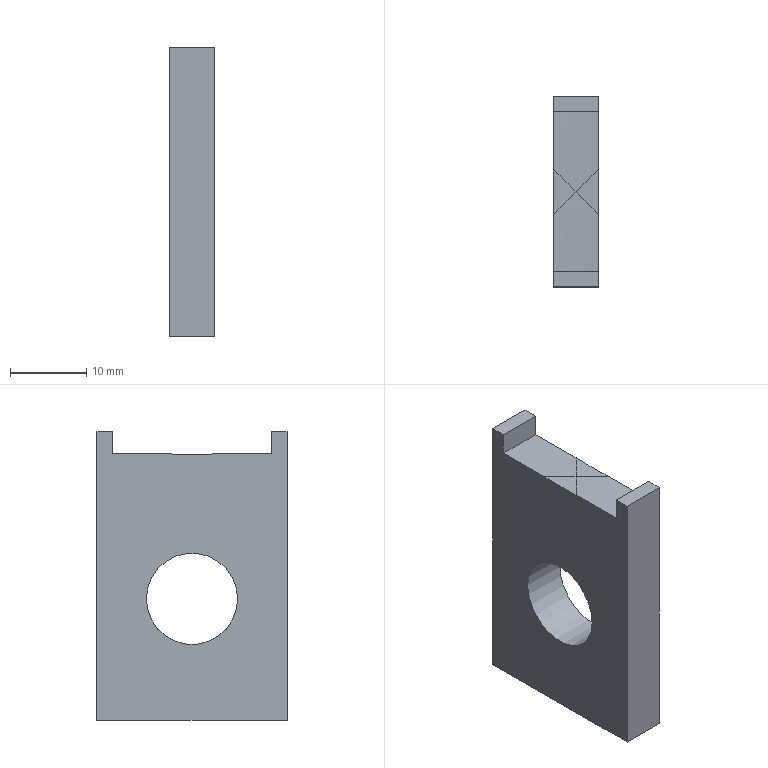Component | NX | PACKING | 1 solid | 14 faces | box 6 x 25 x 38 mm | volume 4646 mm3 | plane 9 | cylinder 5 | commonest cylinder face diameters 152 x4 12 x1
STEP:
#1=CARTESIAN_POINT('',(0.,0.,0.));
#2=DIRECTION('',(0.,0.,1.));
#3=DIRECTION('',(1.,0.,0.));
#4=AXIS2_PLACEMENT_3D('',#1,#2,#3);
#5=CARTESIAN_POINT('',(56.,3.,-75.941));
#6=VERTEX_POINT('',#5);
#7=CARTESIAN_POINT('',(56.,-3.,-75.941));
#8=VERTEX_POINT('',#7);
#9=CARTESIAN_POINT('',(56.,-0.,-0.));
#10=DIRECTION('',(-1.,0.,0.));
#11=DIRECTION('',(0.,-1.,-0.));
#12=AXIS2_PLACEMENT_3D('',#9,#10,#11);
#13=CIRCLE('',#12,76.);
#14=CARTESIAN_POINT('',(62.,-0.,-0.));
#15=DIRECTION('',(-1.,0.,0.));
#16=DIRECTION('',(0.,0.,-1.));
#17=AXIS2_PLACEMENT_3D('',#14,#15,#16);
#18=CYLINDRICAL_SURFACE('',#17,76.);
#19=CARTESIAN_POINT('',(1.571,6.));
#20=DIRECTION('',(1.,0.));
#21=VECTOR('',#20,1.);
#22=LINE('',#19,#21);
#23=(GEOMETRIC_REPRESENTATION_CONTEXT(2)PARAMETRIC_REPRESENTATION_CONTEXT()REPRESENTATION_CONTEXT('',''));
#24=DEFINITIONAL_REPRESENTATION('',(#22),#23);
#25=PCURVE('',#18,#24);
#26=CARTESIAN_POINT('',(56.,-0.,-0.));
#27=DIRECTION('',(-1.,0.,0.));
#28=DIRECTION('',(0.,0.,-1.));
#29=AXIS2_PLACEMENT_3D('',#26,#27,#28);
#30=PLANE('',#29);
#31=CARTESIAN_POINT('',(0.,0.));
#32=DIRECTION('',(0.,1.));
#33=AXIS2_PLACEMENT_2D('',#31,#32);
#34=CIRCLE('',#33,76.);
#35=(GEOMETRIC_REPRESENTATION_CONTEXT(2)PARAMETRIC_REPRESENTATION_CONTEXT()REPRESENTATION_CONTEXT('',''));
#36=DEFINITIONAL_REPRESENTATION('',(#34),#35);
#37=PCURVE('',#30,#36);
#38=SURFACE_CURVE('',#13,(#25,#37),.PCURVE_S1.);
#39=EDGE_CURVE('',#6,#8,#38,.T.);
#40=ORIENTED_EDGE('',*,*,#39,.F.);
#41=CARTESIAN_POINT('',(59.,-0.,-76.));
#42=VERTEX_POINT('',#41);
#43=CARTESIAN_POINT('',(59.,-0.,-0.));
#44=DIRECTION('',(0.7071,0.7071,0.));
#45=DIRECTION('',(-0.7071,0.7071,0.));
#46=AXIS2_PLACEMENT_3D('',#43,#44,#45);
#47=ELLIPSE('',#46,107.48,76.);
#48=CARTESIAN_POINT('',(6.283,3.));
#49=CARTESIAN_POINT('',(6.244,6.));
#50=B_SPLINE_CURVE_WITH_KNOTS('',1,(#48,#49),.UNSPECIFIED.,.F.,.F.,(2,2),(4.712,4.752),.PIECEWISE_BEZIER_KNOTS.);
#51=(GEOMETRIC_REPRESENTATION_CONTEXT(2)PARAMETRIC_REPRESENTATION_CONTEXT()REPRESENTATION_CONTEXT('',''));
#52=DEFINITIONAL_REPRESENTATION('',(#50),#51);
#53=PCURVE('',#18,#52);
#54=CARTESIAN_POINT('',(59.,10.5,-0.));
#55=DIRECTION('',(0.,-1.,0.));
#56=DIRECTION('',(1.,0.,0.));
#57=AXIS2_PLACEMENT_3D('',#54,#55,#56);
#58=CYLINDRICAL_SURFACE('',#57,76.);
#59=CARTESIAN_POINT('',(4.712,10.5));
#60=CARTESIAN_POINT('',(4.673,7.5));
#61=B_SPLINE_CURVE_WITH_KNOTS('',1,(#59,#60),.UNSPECIFIED.,.F.,.F.,(2,2),(4.712,4.752),.PIECEWISE_BEZIER_KNOTS.);
#62=(GEOMETRIC_REPRESENTATION_CONTEXT(2)PARAMETRIC_REPRESENTATION_CONTEXT()REPRESENTATION_CONTEXT('',''));
#63=DEFINITIONAL_REPRESENTATION('',(#61),#62);
#64=PCURVE('',#58,#63);
#65=SURFACE_CURVE('',#47,(#53,#64),.PCURVE_S1.);
#66=EDGE_CURVE('',#42,#6,#65,.T.);
#67=ORIENTED_EDGE('',*,*,#66,.F.);
#68=CARTESIAN_POINT('',(59.,-0.,-0.));
#69=DIRECTION('',(0.7071,-0.7071,0.));
#70=DIRECTION('',(-0.7071,-0.7071,0.));
#71=AXIS2_PLACEMENT_3D('',#68,#69,#70);
#72=ELLIPSE('',#71,107.48,76.);
#73=CARTESIAN_POINT('',(6.323,6.));
#74=CARTESIAN_POINT('',(6.283,3.));
#75=B_SPLINE_CURVE_WITH_KNOTS('',1,(#73,#74),.UNSPECIFIED.,.F.,.F.,(2,2),(1.531,1.571),.PIECEWISE_BEZIER_KNOTS.);
#76=(GEOMETRIC_REPRESENTATION_CONTEXT(2)PARAMETRIC_REPRESENTATION_CONTEXT()REPRESENTATION_CONTEXT('',''));
#77=DEFINITIONAL_REPRESENTATION('',(#75),#76);
#78=PCURVE('',#18,#77);
#79=CARTESIAN_POINT('',(59.,10.5,-0.));
#80=DIRECTION('',(0.,-1.,0.));
#81=DIRECTION('',(1.,0.,0.));
#82=AXIS2_PLACEMENT_3D('',#79,#80,#81);
#83=CYLINDRICAL_SURFACE('',#82,76.);
#84=CARTESIAN_POINT('',(4.673,13.5));
#85=CARTESIAN_POINT('',(4.712,10.5));
#86=B_SPLINE_CURVE_WITH_KNOTS('',1,(#84,#85),.UNSPECIFIED.,.F.,.F.,(2,2),(1.531,1.571),.PIECEWISE_BEZIER_KNOTS.);
#87=(GEOMETRIC_REPRESENTATION_CONTEXT(2)PARAMETRIC_REPRESENTATION_CONTEXT()REPRESENTATION_CONTEXT('',''));
#88=DEFINITIONAL_REPRESENTATION('',(#86),#87);
#89=PCURVE('',#83,#88);
#90=SURFACE_CURVE('',#72,(#78,#89),.PCURVE_S1.);
#91=EDGE_CURVE('',#8,#42,#90,.T.);
#92=ORIENTED_EDGE('',*,*,#91,.F.);
#93=EDGE_LOOP('',(#40,#67,#92));
#94=FACE_BOUND('',#93,.F.);
#95=ADVANCED_FACE('',(#94),#18,.F.);
#96=CARTESIAN_POINT('',(56.,12.5,-111.));
#97=VERTEX_POINT('',#96);
#98=CARTESIAN_POINT('',(56.,12.5,-73.));
#99=VERTEX_POINT('',#98);
#100=CARTESIAN_POINT('',(56.,12.5,-111.));
#101=DIRECTION('',(0.,0.,1.));
#102=VECTOR('',#101,1.);
#103=LINE('',#100,#102);
#104=CARTESIAN_POINT('',(62.,12.5,-111.));
#105=DIRECTION('',(0.,-1.,0.));
#106=DIRECTION('',(0.,-0.,-1.));
#107=AXIS2_PLACEMENT_3D('',#104,#105,#106);
#108=PLANE('',#107);
#109=CARTESIAN_POINT('',(0.,-6.));
#110=DIRECTION('',(-1.,0.));
#111=VECTOR('',#110,1.);
#112=LINE('',#109,#111);
#113=(GEOMETRIC_REPRESENTATION_CONTEXT(2)PARAMETRIC_REPRESENTATION_CONTEXT()REPRESENTATION_CONTEXT('',''));
#114=DEFINITIONAL_REPRESENTATION('',(#112),#113);
#115=PCURVE('',#108,#114);
#116=CARTESIAN_POINT('',(111.,-12.5));
#117=DIRECTION('',(-1.,-0.));
#118=VECTOR('',#117,1.);
#119=LINE('',#116,#118);
#120=(GEOMETRIC_REPRESENTATION_CONTEXT(2)PARAMETRIC_REPRESENTATION_CONTEXT()REPRESENTATION_CONTEXT('',''));
#121=DEFINITIONAL_REPRESENTATION('',(#119),#120);
#122=PCURVE('',#30,#121);
#123=SURFACE_CURVE('',#103,(#115,#122),.PCURVE_S1.);
#124=EDGE_CURVE('',#97,#99,#123,.T.);
#125=ORIENTED_EDGE('',*,*,#124,.T.);
#126=CARTESIAN_POINT('',(62.,12.5,-73.));
#127=VERTEX_POINT('',#126);
#128=CARTESIAN_POINT('',(62.,12.5,-73.));
#129=DIRECTION('',(-1.,0.,0.));
#130=VECTOR('',#129,1.);
#131=LINE('',#128,#130);
#132=CARTESIAN_POINT('',(-38.,0.));
#133=DIRECTION('',(0.,-1.));
#134=VECTOR('',#133,1.);
#135=LINE('',#132,#134);
#136=(GEOMETRIC_REPRESENTATION_CONTEXT(2)PARAMETRIC_REPRESENTATION_CONTEXT()REPRESENTATION_CONTEXT('',''));
#137=DEFINITIONAL_REPRESENTATION('',(#135),#136);
#138=PCURVE('',#108,#137);
#139=CARTESIAN_POINT('',(62.,12.5,-73.));
#140=DIRECTION('',(0.,-0.,-1.));
#141=DIRECTION('',(0.,1.,-0.));
#142=AXIS2_PLACEMENT_3D('',#139,#140,#141);
#143=PLANE('',#142);
#144=CARTESIAN_POINT('',(0.,0.));
#145=DIRECTION('',(0.,-1.));
#146=VECTOR('',#145,1.);
#147=LINE('',#144,#146);
#148=(GEOMETRIC_REPRESENTATION_CONTEXT(2)PARAMETRIC_REPRESENTATION_CONTEXT()REPRESENTATION_CONTEXT('',''));
#149=DEFINITIONAL_REPRESENTATION('',(#147),#148);
#150=PCURVE('',#143,#149);
#151=SURFACE_CURVE('',#131,(#138,#150),.PCURVE_S1.);
#152=EDGE_CURVE('',#127,#99,#151,.T.);
#153=ORIENTED_EDGE('',*,*,#152,.F.);
#154=CARTESIAN_POINT('',(62.,12.5,-111.));
#155=VERTEX_POINT('',#154);
#156=CARTESIAN_POINT('',(62.,12.5,-111.));
#157=DIRECTION('',(0.,0.,1.));
#158=VECTOR('',#157,1.);
#159=LINE('',#156,#158);
#160=CARTESIAN_POINT('',(0.,0.));
#161=DIRECTION('',(-1.,0.));
#162=VECTOR('',#161,1.);
#163=LINE('',#160,#162);
#164=(GEOMETRIC_REPRESENTATION_CONTEXT(2)PARAMETRIC_REPRESENTATION_CONTEXT()REPRESENTATION_CONTEXT('',''));
#165=DEFINITIONAL_REPRESENTATION('',(#163),#164);
#166=PCURVE('',#108,#165);
#167=CARTESIAN_POINT('',(62.,-0.,-0.));
#168=DIRECTION('',(-1.,0.,0.));
#169=DIRECTION('',(0.,0.,-1.));
#170=AXIS2_PLACEMENT_3D('',#167,#168,#169);
#171=PLANE('',#170);
#172=CARTESIAN_POINT('',(111.,-12.5));
#173=DIRECTION('',(-1.,-0.));
#174=VECTOR('',#173,1.);
#175=LINE('',#172,#174);
#176=(GEOMETRIC_REPRESENTATION_CONTEXT(2)PARAMETRIC_REPRESENTATION_CONTEXT()REPRESENTATION_CONTEXT('',''));
#177=DEFINITIONAL_REPRESENTATION('',(#175),#176);
#178=PCURVE('',#171,#177);
#179=SURFACE_CURVE('',#159,(#166,#178),.PCURVE_S1.);
#180=EDGE_CURVE('',#155,#127,#179,.T.);
#181=ORIENTED_EDGE('',*,*,#180,.F.);
#182=CARTESIAN_POINT('',(62.,12.5,-111.));
#183=DIRECTION('',(-1.,0.,0.));
#184=VECTOR('',#183,1.);
#185=LINE('',#182,#184);
#186=CARTESIAN_POINT('',(0.,0.));
#187=DIRECTION('',(0.,-1.));
#188=VECTOR('',#187,1.);
#189=LINE('',#186,#188);
#190=(GEOMETRIC_REPRESENTATION_CONTEXT(2)PARAMETRIC_REPRESENTATION_CONTEXT()REPRESENTATION_CONTEXT('',''));
#191=DEFINITIONAL_REPRESENTATION('',(#189),#190);
#192=PCURVE('',#108,#191);
#193=CARTESIAN_POINT('',(62.,-0.,-111.));
#194=DIRECTION('',(0.,0.,1.));
#195=DIRECTION('',(-1.,0.,0.));
#196=AXIS2_PLACEMENT_3D('',#193,#194,#195);
#197=PLANE('',#196);
#198=CARTESIAN_POINT('',(0.,-12.5));
#199=DIRECTION('',(1.,0.));
#200=VECTOR('',#199,1.);
#201=LINE('',#198,#200);
#202=(GEOMETRIC_REPRESENTATION_CONTEXT(2)PARAMETRIC_REPRESENTATION_CONTEXT()REPRESENTATION_CONTEXT('',''));
#203=DEFINITIONAL_REPRESENTATION('',(#201),#202);
#204=PCURVE('',#197,#203);
#205=SURFACE_CURVE('',#185,(#192,#204),.PCURVE_S1.);
#206=EDGE_CURVE('',#155,#97,#205,.T.);
#207=ORIENTED_EDGE('',*,*,#206,.T.);
#208=EDGE_LOOP('',(#125,#153,#181,#207));
#209=FACE_BOUND('',#208,.T.);
#210=ADVANCED_FACE('',(#209),#108,.F.);
#211=CARTESIAN_POINT('',(56.,10.5,-73.));
#212=VERTEX_POINT('',#211);
#213=CARTESIAN_POINT('',(56.,12.5,-73.));
#214=DIRECTION('',(0.,-1.,0.));
#215=VECTOR('',#214,1.);
#216=LINE('',#213,#215);
#217=CARTESIAN_POINT('',(0.,-6.));
#218=DIRECTION('',(-1.,0.));
#219=VECTOR('',#218,1.);
#220=LINE('',#217,#219);
#221=(GEOMETRIC_REPRESENTATION_CONTEXT(2)PARAMETRIC_REPRESENTATION_CONTEXT()REPRESENTATION_CONTEXT('',''));
#222=DEFINITIONAL_REPRESENTATION('',(#220),#221);
#223=PCURVE('',#143,#222);
#224=CARTESIAN_POINT('',(73.,-12.5));
#225=DIRECTION('',(-0.,1.));
#226=VECTOR('',#225,1.);
#227=LINE('',#224,#226);
#228=(GEOMETRIC_REPRESENTATION_CONTEXT(2)PARAMETRIC_REPRESENTATION_CONTEXT()REPRESENTATION_CONTEXT('',''));
#229=DEFINITIONAL_REPRESENTATION('',(#227),#228);
#230=PCURVE('',#30,#229);
#231=SURFACE_CURVE('',#216,(#223,#230),.PCURVE_S1.);
#232=EDGE_CURVE('',#99,#212,#231,.T.);
#233=ORIENTED_EDGE('',*,*,#232,.T.);
#234=CARTESIAN_POINT('',(62.,10.5,-73.));
#235=VERTEX_POINT('',#234);
#236=CARTESIAN_POINT('',(62.,10.5,-73.));
#237=DIRECTION('',(-1.,0.,0.));
#238=VECTOR('',#237,1.);
#239=LINE('',#236,#238);
#240=CARTESIAN_POINT('',(-2.,0.));
#241=DIRECTION('',(0.,-1.));
#242=VECTOR('',#241,1.);
#243=LINE('',#240,#242);
#244=(GEOMETRIC_REPRESENTATION_CONTEXT(2)PARAMETRIC_REPRESENTATION_CONTEXT()REPRESENTATION_CONTEXT('',''));
#245=DEFINITIONAL_REPRESENTATION('',(#243),#244);
#246=PCURVE('',#143,#245);
#247=CARTESIAN_POINT('',(62.,10.5,-73.));
#248=DIRECTION('',(0.,1.,0.));
#249=DIRECTION('',(0.,0.,1.));
#250=AXIS2_PLACEMENT_3D('',#247,#248,#249);
#251=PLANE('',#250);
#252=CARTESIAN_POINT('',(0.,0.));
#253=DIRECTION('',(0.,-1.));
#254=VECTOR('',#253,1.);
#255=LINE('',#252,#254);
#256=(GEOMETRIC_REPRESENTATION_CONTEXT(2)PARAMETRIC_REPRESENTATION_CONTEXT()REPRESENTATION_CONTEXT('',''));
#257=DEFINITIONAL_REPRESENTATION('',(#255),#256);
#258=PCURVE('',#251,#257);
#259=SURFACE_CURVE('',#239,(#246,#258),.PCURVE_S1.);
#260=EDGE_CURVE('',#235,#212,#259,.T.);
#261=ORIENTED_EDGE('',*,*,#260,.F.);
#262=CARTESIAN_POINT('',(62.,12.5,-73.));
#263=DIRECTION('',(0.,-1.,0.));
#264=VECTOR('',#263,1.);
#265=LINE('',#262,#264);
#266=CARTESIAN_POINT('',(0.,0.));
#267=DIRECTION('',(-1.,0.));
#268=VECTOR('',#267,1.);
#269=LINE('',#266,#268);
#270=(GEOMETRIC_REPRESENTATION_CONTEXT(2)PARAMETRIC_REPRESENTATION_CONTEXT()REPRESENTATION_CONTEXT('',''));
#271=DEFINITIONAL_REPRESENTATION('',(#269),#270);
#272=PCURVE('',#143,#271);
#273=CARTESIAN_POINT('',(73.,-12.5));
#274=DIRECTION('',(-0.,1.));
#275=VECTOR('',#274,1.);
#276=LINE('',#273,#275);
#277=(GEOMETRIC_REPRESENTATION_CONTEXT(2)PARAMETRIC_REPRESENTATION_CONTEXT()REPRESENTATION_CONTEXT('',''));
#278=DEFINITIONAL_REPRESENTATION('',(#276),#277);
#279=PCURVE('',#171,#278);
#280=SURFACE_CURVE('',#265,(#272,#279),.PCURVE_S1.);
#281=EDGE_CURVE('',#127,#235,#280,.T.);
#282=ORIENTED_EDGE('',*,*,#281,.F.);
#283=ORIENTED_EDGE('',*,*,#152,.T.);
#284=EDGE_LOOP('',(#233,#261,#282,#283));
#285=FACE_BOUND('',#284,.T.);
#286=ADVANCED_FACE('',(#285),#143,.F.);
#287=CARTESIAN_POINT('',(56.,10.5,-75.941));
#288=VERTEX_POINT('',#287);
#289=CARTESIAN_POINT('',(56.,10.5,-73.));
#290=DIRECTION('',(0.,0.,-1.));
#291=VECTOR('',#290,1.);
#292=LINE('',#289,#291);
#293=CARTESIAN_POINT('',(0.,-6.));
#294=DIRECTION('',(-1.,0.));
#295=VECTOR('',#294,1.);
#296=LINE('',#293,#295);
#297=(GEOMETRIC_REPRESENTATION_CONTEXT(2)PARAMETRIC_REPRESENTATION_CONTEXT()REPRESENTATION_CONTEXT('',''));
#298=DEFINITIONAL_REPRESENTATION('',(#296),#297);
#299=PCURVE('',#251,#298);
#300=CARTESIAN_POINT('',(73.,-10.5));
#301=DIRECTION('',(1.,0.));
#302=VECTOR('',#301,1.);
#303=LINE('',#300,#302);
#304=(GEOMETRIC_REPRESENTATION_CONTEXT(2)PARAMETRIC_REPRESENTATION_CONTEXT()REPRESENTATION_CONTEXT('',''));
#305=DEFINITIONAL_REPRESENTATION('',(#303),#304);
#306=PCURVE('',#30,#305);
#307=SURFACE_CURVE('',#292,(#299,#306),.PCURVE_S1.);
#308=EDGE_CURVE('',#212,#288,#307,.T.);
#309=ORIENTED_EDGE('',*,*,#308,.T.);
#310=CARTESIAN_POINT('',(62.,10.5,-75.941));
#311=VERTEX_POINT('',#310);
#312=CARTESIAN_POINT('',(59.,10.5,-0.));
#313=DIRECTION('',(0.,-1.,0.));
#314=DIRECTION('',(1.,0.,0.));
#315=AXIS2_PLACEMENT_3D('',#312,#313,#314);
#316=CIRCLE('',#315,76.);
#317=CARTESIAN_POINT('',(73.,73.));
#318=CARTESIAN_POINT('',(204.636,73.));
#319=CARTESIAN_POINT('',(138.818,-41.));
#320=CARTESIAN_POINT('',(73.,-155.));
#321=CARTESIAN_POINT('',(7.182,-41.));
#322=CARTESIAN_POINT('',(-58.636,73.));
#323=CARTESIAN_POINT('',(73.,73.));
#324=(BOUNDED_CURVE()B_SPLINE_CURVE(2,(#317,#318,#319,#320,#321,#322,#323),.UNSPECIFIED.,.T.,.F.)B_SPLINE_CURVE_WITH_KNOTS((1,2,2,2,2,1),(-2.094,0.,2.094,4.189,6.283,8.378),.UNSPECIFIED.)CURVE()GEOMETRIC_REPRESENTATION_ITEM()RATIONAL_B_SPLINE_CURVE((1.,0.5,1.,0.5,1.,0.5,1.))REPRESENTATION_ITEM(''));
#325=(GEOMETRIC_REPRESENTATION_CONTEXT(2)PARAMETRIC_REPRESENTATION_CONTEXT()REPRESENTATION_CONTEXT('',''));
#326=DEFINITIONAL_REPRESENTATION('',(#324),#325);
#327=PCURVE('',#251,#326);
#328=CARTESIAN_POINT('',(0.,0.));
#329=DIRECTION('',(1.,0.));
#330=VECTOR('',#329,1.);
#331=LINE('',#328,#330);
#332=(GEOMETRIC_REPRESENTATION_CONTEXT(2)PARAMETRIC_REPRESENTATION_CONTEXT()REPRESENTATION_CONTEXT('',''));
#333=DEFINITIONAL_REPRESENTATION('',(#331),#332);
#334=PCURVE('',#58,#333);
#335=SURFACE_CURVE('',#316,(#327,#334),.PCURVE_S1.);
#336=EDGE_CURVE('',#288,#311,#335,.T.);
#337=ORIENTED_EDGE('',*,*,#336,.T.);
#338=CARTESIAN_POINT('',(62.,10.5,-73.));
#339=DIRECTION('',(0.,0.,-1.));
#340=VECTOR('',#339,1.);
#341=LINE('',#338,#340);
#342=CARTESIAN_POINT('',(0.,0.));
#343=DIRECTION('',(-1.,0.));
#344=VECTOR('',#343,1.);
#345=LINE('',#342,#344);
#346=(GEOMETRIC_REPRESENTATION_CONTEXT(2)PARAMETRIC_REPRESENTATION_CONTEXT()REPRESENTATION_CONTEXT('',''));
#347=DEFINITIONAL_REPRESENTATION('',(#345),#346);
#348=PCURVE('',#251,#347);
#349=CARTESIAN_POINT('',(73.,-10.5));
#350=DIRECTION('',(1.,0.));
#351=VECTOR('',#350,1.);
#352=LINE('',#349,#351);
#353=(GEOMETRIC_REPRESENTATION_CONTEXT(2)PARAMETRIC_REPRESENTATION_CONTEXT()REPRESENTATION_CONTEXT('',''));
#354=DEFINITIONAL_REPRESENTATION('',(#352),#353);
#355=PCURVE('',#171,#354);
#356=SURFACE_CURVE('',#341,(#348,#355),.PCURVE_S1.);
#357=EDGE_CURVE('',#235,#311,#356,.T.);
#358=ORIENTED_EDGE('',*,*,#357,.F.);
#359=ORIENTED_EDGE('',*,*,#260,.T.);
#360=EDGE_LOOP('',(#309,#337,#358,#359));
#361=FACE_BOUND('',#360,.T.);
#362=ADVANCED_FACE('',(#361),#251,.F.);
#363=CARTESIAN_POINT('',(62.,3.,-75.941));
#364=VERTEX_POINT('',#363);
#365=CARTESIAN_POINT('',(62.,-3.,-75.941));
#366=VERTEX_POINT('',#365);
#367=CARTESIAN_POINT('',(62.,-0.,-0.));
#368=DIRECTION('',(-1.,0.,0.));
#369=DIRECTION('',(0.,-1.,-0.));
#370=AXIS2_PLACEMENT_3D('',#367,#368,#369);
#371=CIRCLE('',#370,76.);
#372=CARTESIAN_POINT('',(62.,-0.,-0.));
#373=DIRECTION('',(-1.,0.,0.));
#374=DIRECTION('',(0.,0.,-1.));
#375=AXIS2_PLACEMENT_3D('',#372,#373,#374);
#376=CYLINDRICAL_SURFACE('',#375,76.);
#377=CARTESIAN_POINT('',(1.571,0.));
#378=DIRECTION('',(1.,0.));
#379=VECTOR('',#378,1.);
#380=LINE('',#377,#379);
#381=(GEOMETRIC_REPRESENTATION_CONTEXT(2)PARAMETRIC_REPRESENTATION_CONTEXT()REPRESENTATION_CONTEXT('',''));
#382=DEFINITIONAL_REPRESENTATION('',(#380),#381);
#383=PCURVE('',#376,#382);
#384=CARTESIAN_POINT('',(0.,0.));
#385=DIRECTION('',(0.,1.));
#386=AXIS2_PLACEMENT_2D('',#384,#385);
#387=CIRCLE('',#386,76.);
#388=(GEOMETRIC_REPRESENTATION_CONTEXT(2)PARAMETRIC_REPRESENTATION_CONTEXT()REPRESENTATION_CONTEXT('',''));
#389=DEFINITIONAL_REPRESENTATION('',(#387),#388);
#390=PCURVE('',#171,#389);
#391=SURFACE_CURVE('',#371,(#383,#390),.PCURVE_S1.);
#392=EDGE_CURVE('',#364,#366,#391,.T.);
#393=ORIENTED_EDGE('',*,*,#392,.T.);
#394=CARTESIAN_POINT('',(59.,-0.,-0.));
#395=DIRECTION('',(-0.7071,-0.7071,0.));
#396=DIRECTION('',(-0.7071,0.7071,0.));
#397=AXIS2_PLACEMENT_3D('',#394,#395,#396);
#398=ELLIPSE('',#397,107.48,76.);
#399=CARTESIAN_POINT('',(6.283,3.));
#400=CARTESIAN_POINT('',(6.323,-0.));
#401=B_SPLINE_CURVE_WITH_KNOTS('',1,(#399,#400),.UNSPECIFIED.,.F.,.F.,(2,2),(1.571,1.61),.PIECEWISE_BEZIER_KNOTS.);
#402=(GEOMETRIC_REPRESENTATION_CONTEXT(2)PARAMETRIC_REPRESENTATION_CONTEXT()REPRESENTATION_CONTEXT('',''));
#403=DEFINITIONAL_REPRESENTATION('',(#401),#402);
#404=PCURVE('',#376,#403);
#405=CARTESIAN_POINT('',(4.712,10.5));
#406=CARTESIAN_POINT('',(4.752,13.5));
#407=B_SPLINE_CURVE_WITH_KNOTS('',1,(#405,#406),.UNSPECIFIED.,.F.,.F.,(2,2),(1.571,1.61),.PIECEWISE_BEZIER_KNOTS.);
#408=(GEOMETRIC_REPRESENTATION_CONTEXT(2)PARAMETRIC_REPRESENTATION_CONTEXT()REPRESENTATION_CONTEXT('',''));
#409=DEFINITIONAL_REPRESENTATION('',(#407),#408);
#410=PCURVE('',#83,#409);
#411=SURFACE_CURVE('',#398,(#404,#410),.PCURVE_S1.);
#412=EDGE_CURVE('',#42,#366,#411,.T.);
#413=ORIENTED_EDGE('',*,*,#412,.F.);
#414=CARTESIAN_POINT('',(59.,-0.,-0.));
#415=DIRECTION('',(-0.7071,0.7071,0.));
#416=DIRECTION('',(-0.7071,-0.7071,0.));
#417=AXIS2_PLACEMENT_3D('',#414,#415,#416);
#418=ELLIPSE('',#417,107.48,76.);
#419=CARTESIAN_POINT('',(6.244,-0.));
#420=CARTESIAN_POINT('',(6.283,3.));
#421=B_SPLINE_CURVE_WITH_KNOTS('',1,(#419,#420),.UNSPECIFIED.,.F.,.F.,(2,2),(4.673,4.712),.PIECEWISE_BEZIER_KNOTS.);
#422=(GEOMETRIC_REPRESENTATION_CONTEXT(2)PARAMETRIC_REPRESENTATION_CONTEXT()REPRESENTATION_CONTEXT('',''));
#423=DEFINITIONAL_REPRESENTATION('',(#421),#422);
#424=PCURVE('',#376,#423);
#425=CARTESIAN_POINT('',(4.752,7.5));
#426=CARTESIAN_POINT('',(4.712,10.5));
#427=B_SPLINE_CURVE_WITH_KNOTS('',1,(#425,#426),.UNSPECIFIED.,.F.,.F.,(2,2),(4.673,4.712),.PIECEWISE_BEZIER_KNOTS.);
#428=(GEOMETRIC_REPRESENTATION_CONTEXT(2)PARAMETRIC_REPRESENTATION_CONTEXT()REPRESENTATION_CONTEXT('',''));
#429=DEFINITIONAL_REPRESENTATION('',(#427),#428);
#430=PCURVE('',#58,#429);
#431=SURFACE_CURVE('',#418,(#424,#430),.PCURVE_S1.);
#432=EDGE_CURVE('',#364,#42,#431,.T.);
#433=ORIENTED_EDGE('',*,*,#432,.F.);
#434=EDGE_LOOP('',(#393,#413,#433));
#435=FACE_BOUND('',#434,.F.);
#436=ADVANCED_FACE('',(#435),#376,.F.);
#437=CARTESIAN_POINT('',(56.,-10.5,-75.941));
#438=VERTEX_POINT('',#437);
#439=CARTESIAN_POINT('',(56.,-10.5,-73.));
#440=VERTEX_POINT('',#439);
#441=CARTESIAN_POINT('',(56.,-10.5,-75.271));
#442=DIRECTION('',(0.,0.,1.));
#443=VECTOR('',#442,1.);
#444=LINE('',#441,#443);
#445=CARTESIAN_POINT('',(62.,-10.5,-75.271));
#446=DIRECTION('',(0.,-1.,0.));
#447=DIRECTION('',(0.,0.,-1.));
#448=AXIS2_PLACEMENT_3D('',#445,#446,#447);
#449=PLANE('',#448);
#450=CARTESIAN_POINT('',(0.,-6.));
#451=DIRECTION('',(-1.,0.));
#452=VECTOR('',#451,1.);
#453=LINE('',#450,#452);
#454=(GEOMETRIC_REPRESENTATION_CONTEXT(2)PARAMETRIC_REPRESENTATION_CONTEXT()REPRESENTATION_CONTEXT('',''));
#455=DEFINITIONAL_REPRESENTATION('',(#453),#454);
#456=PCURVE('',#449,#455);
#457=CARTESIAN_POINT('',(75.271,10.5));
#458=DIRECTION('',(-1.,0.));
#459=VECTOR('',#458,1.);
#460=LINE('',#457,#459);
#461=(GEOMETRIC_REPRESENTATION_CONTEXT(2)PARAMETRIC_REPRESENTATION_CONTEXT()REPRESENTATION_CONTEXT('',''));
#462=DEFINITIONAL_REPRESENTATION('',(#460),#461);
#463=PCURVE('',#30,#462);
#464=SURFACE_CURVE('',#444,(#456,#463),.PCURVE_S1.);
#465=EDGE_CURVE('',#438,#440,#464,.T.);
#466=ORIENTED_EDGE('',*,*,#465,.T.);
#467=CARTESIAN_POINT('',(62.,-10.5,-73.));
#468=VERTEX_POINT('',#467);
#469=CARTESIAN_POINT('',(62.,-10.5,-73.));
#470=DIRECTION('',(-1.,0.,0.));
#471=VECTOR('',#470,1.);
#472=LINE('',#469,#471);
#473=CARTESIAN_POINT('',(-2.271,0.));
#474=DIRECTION('',(0.,-1.));
#475=VECTOR('',#474,1.);
#476=LINE('',#473,#475);
#477=(GEOMETRIC_REPRESENTATION_CONTEXT(2)PARAMETRIC_REPRESENTATION_CONTEXT()REPRESENTATION_CONTEXT('',''));
#478=DEFINITIONAL_REPRESENTATION('',(#476),#477);
#479=PCURVE('',#449,#478);
#480=CARTESIAN_POINT('',(62.,-10.5,-73.));
#481=DIRECTION('',(0.,0.,-1.));
#482=DIRECTION('',(0.,1.,0.));
#483=AXIS2_PLACEMENT_3D('',#480,#481,#482);
#484=PLANE('',#483);
#485=CARTESIAN_POINT('',(0.,0.));
#486=DIRECTION('',(0.,-1.));
#487=VECTOR('',#486,1.);
#488=LINE('',#485,#487);
#489=(GEOMETRIC_REPRESENTATION_CONTEXT(2)PARAMETRIC_REPRESENTATION_CONTEXT()REPRESENTATION_CONTEXT('',''));
#490=DEFINITIONAL_REPRESENTATION('',(#488),#489);
#491=PCURVE('',#484,#490);
#492=SURFACE_CURVE('',#472,(#479,#491),.PCURVE_S1.);
#493=EDGE_CURVE('',#468,#440,#492,.T.);
#494=ORIENTED_EDGE('',*,*,#493,.F.);
#495=CARTESIAN_POINT('',(62.,-10.5,-75.941));
#496=VERTEX_POINT('',#495);
#497=CARTESIAN_POINT('',(62.,-10.5,-75.271));
#498=DIRECTION('',(0.,0.,1.));
#499=VECTOR('',#498,1.);
#500=LINE('',#497,#499);
#501=CARTESIAN_POINT('',(0.,0.));
#502=DIRECTION('',(-1.,0.));
#503=VECTOR('',#502,1.);
#504=LINE('',#501,#503);
#505=(GEOMETRIC_REPRESENTATION_CONTEXT(2)PARAMETRIC_REPRESENTATION_CONTEXT()REPRESENTATION_CONTEXT('',''));
#506=DEFINITIONAL_REPRESENTATION('',(#504),#505);
#507=PCURVE('',#449,#506);
#508=CARTESIAN_POINT('',(75.271,10.5));
#509=DIRECTION('',(-1.,0.));
#510=VECTOR('',#509,1.);
#511=LINE('',#508,#510);
#512=(GEOMETRIC_REPRESENTATION_CONTEXT(2)PARAMETRIC_REPRESENTATION_CONTEXT()REPRESENTATION_CONTEXT('',''));
#513=DEFINITIONAL_REPRESENTATION('',(#511),#512);
#514=PCURVE('',#171,#513);
#515=SURFACE_CURVE('',#500,(#507,#514),.PCURVE_S1.);
#516=EDGE_CURVE('',#496,#468,#515,.T.);
#517=ORIENTED_EDGE('',*,*,#516,.F.);
#518=CARTESIAN_POINT('',(59.,-10.5,-0.));
#519=DIRECTION('',(0.,1.,0.));
#520=DIRECTION('',(1.,0.,0.));
#521=AXIS2_PLACEMENT_3D('',#518,#519,#520);
#522=CIRCLE('',#521,76.);
#523=CARTESIAN_POINT('',(-75.271,73.));
#524=CARTESIAN_POINT('',(56.365,73.));
#525=CARTESIAN_POINT('',(-9.453,-41.));
#526=CARTESIAN_POINT('',(-75.271,-155.));
#527=CARTESIAN_POINT('',(-141.089,-41.));
#528=CARTESIAN_POINT('',(-206.907,73.));
#529=CARTESIAN_POINT('',(-75.271,73.));
#530=(BOUNDED_CURVE()B_SPLINE_CURVE(2,(#523,#524,#525,#526,#527,#528,#529),.UNSPECIFIED.,.T.,.F.)B_SPLINE_CURVE_WITH_KNOTS((1,2,2,2,2,1),(-2.094,0.,2.094,4.189,6.283,8.378),.UNSPECIFIED.)CURVE()GEOMETRIC_REPRESENTATION_ITEM()RATIONAL_B_SPLINE_CURVE((1.,0.5,1.,0.5,1.,0.5,1.))REPRESENTATION_ITEM(''));
#531=(GEOMETRIC_REPRESENTATION_CONTEXT(2)PARAMETRIC_REPRESENTATION_CONTEXT()REPRESENTATION_CONTEXT('',''));
#532=DEFINITIONAL_REPRESENTATION('',(#530),#531);
#533=PCURVE('',#449,#532);
#534=CARTESIAN_POINT('',(6.283,21.));
#535=DIRECTION('',(-1.,0.));
#536=VECTOR('',#535,1.);
#537=LINE('',#534,#536);
#538=(GEOMETRIC_REPRESENTATION_CONTEXT(2)PARAMETRIC_REPRESENTATION_CONTEXT()REPRESENTATION_CONTEXT('',''));
#539=DEFINITIONAL_REPRESENTATION('',(#537),#538);
#540=PCURVE('',#83,#539);
#541=SURFACE_CURVE('',#522,(#533,#540),.PCURVE_S1.);
#542=EDGE_CURVE('',#496,#438,#541,.T.);
#543=ORIENTED_EDGE('',*,*,#542,.T.);
#544=EDGE_LOOP('',(#466,#494,#517,#543));
#545=FACE_BOUND('',#544,.T.);
#546=ADVANCED_FACE('',(#545),#449,.F.);
#547=CARTESIAN_POINT('',(56.,-12.5,-73.));
#548=VERTEX_POINT('',#547);
#549=CARTESIAN_POINT('',(56.,-10.5,-73.));
#550=DIRECTION('',(0.,-1.,-0.));
#551=VECTOR('',#550,1.);
#552=LINE('',#549,#551);
#553=CARTESIAN_POINT('',(0.,-6.));
#554=DIRECTION('',(-1.,0.));
#555=VECTOR('',#554,1.);
#556=LINE('',#553,#555);
#557=(GEOMETRIC_REPRESENTATION_CONTEXT(2)PARAMETRIC_REPRESENTATION_CONTEXT()REPRESENTATION_CONTEXT('',''));
#558=DEFINITIONAL_REPRESENTATION('',(#556),#557);
#559=PCURVE('',#484,#558);
#560=CARTESIAN_POINT('',(73.,10.5));
#561=DIRECTION('',(0.,1.));
#562=VECTOR('',#561,1.);
#563=LINE('',#560,#562);
#564=(GEOMETRIC_REPRESENTATION_CONTEXT(2)PARAMETRIC_REPRESENTATION_CONTEXT()REPRESENTATION_CONTEXT('',''));
#565=DEFINITIONAL_REPRESENTATION('',(#563),#564);
#566=PCURVE('',#30,#565);
#567=SURFACE_CURVE('',#552,(#559,#566),.PCURVE_S1.);
#568=EDGE_CURVE('',#440,#548,#567,.T.);
#569=ORIENTED_EDGE('',*,*,#568,.T.);
#570=CARTESIAN_POINT('',(62.,-12.5,-73.));
#571=VERTEX_POINT('',#570);
#572=CARTESIAN_POINT('',(62.,-12.5,-73.));
#573=DIRECTION('',(-1.,0.,0.));
#574=VECTOR('',#573,1.);
#575=LINE('',#572,#574);
#576=CARTESIAN_POINT('',(-2.,0.));
#577=DIRECTION('',(0.,-1.));
#578=VECTOR('',#577,1.);
#579=LINE('',#576,#578);
#580=(GEOMETRIC_REPRESENTATION_CONTEXT(2)PARAMETRIC_REPRESENTATION_CONTEXT()REPRESENTATION_CONTEXT('',''));
#581=DEFINITIONAL_REPRESENTATION('',(#579),#580);
#582=PCURVE('',#484,#581);
#583=CARTESIAN_POINT('',(62.,-12.5,-73.));
#584=DIRECTION('',(0.,1.,0.));
#585=DIRECTION('',(0.,-0.,1.));
#586=AXIS2_PLACEMENT_3D('',#583,#584,#585);
#587=PLANE('',#586);
#588=CARTESIAN_POINT('',(0.,0.));
#589=DIRECTION('',(0.,-1.));
#590=VECTOR('',#589,1.);
#591=LINE('',#588,#590);
#592=(GEOMETRIC_REPRESENTATION_CONTEXT(2)PARAMETRIC_REPRESENTATION_CONTEXT()REPRESENTATION_CONTEXT('',''));
#593=DEFINITIONAL_REPRESENTATION('',(#591),#592);
#594=PCURVE('',#587,#593);
#595=SURFACE_CURVE('',#575,(#582,#594),.PCURVE_S1.);
#596=EDGE_CURVE('',#571,#548,#595,.T.);
#597=ORIENTED_EDGE('',*,*,#596,.F.);
#598=CARTESIAN_POINT('',(62.,-10.5,-73.));
#599=DIRECTION('',(0.,-1.,-0.));
#600=VECTOR('',#599,1.);
#601=LINE('',#598,#600);
#602=CARTESIAN_POINT('',(0.,0.));
#603=DIRECTION('',(-1.,0.));
#604=VECTOR('',#603,1.);
#605=LINE('',#602,#604);
#606=(GEOMETRIC_REPRESENTATION_CONTEXT(2)PARAMETRIC_REPRESENTATION_CONTEXT()REPRESENTATION_CONTEXT('',''));
#607=DEFINITIONAL_REPRESENTATION('',(#605),#606);
#608=PCURVE('',#484,#607);
#609=CARTESIAN_POINT('',(73.,10.5));
#610=DIRECTION('',(0.,1.));
#611=VECTOR('',#610,1.);
#612=LINE('',#609,#611);
#613=(GEOMETRIC_REPRESENTATION_CONTEXT(2)PARAMETRIC_REPRESENTATION_CONTEXT()REPRESENTATION_CONTEXT('',''));
#614=DEFINITIONAL_REPRESENTATION('',(#612),#613);
#615=PCURVE('',#171,#614);
#616=SURFACE_CURVE('',#601,(#608,#615),.PCURVE_S1.);
#617=EDGE_CURVE('',#468,#571,#616,.T.);
#618=ORIENTED_EDGE('',*,*,#617,.F.);
#619=ORIENTED_EDGE('',*,*,#493,.T.);
#620=EDGE_LOOP('',(#569,#597,#618,#619));
#621=FACE_BOUND('',#620,.T.);
#622=ADVANCED_FACE('',(#621),#484,.F.);
#623=CARTESIAN_POINT('',(56.,-12.5,-111.));
#624=VERTEX_POINT('',#623);
#625=CARTESIAN_POINT('',(56.,-12.5,-73.));
#626=DIRECTION('',(0.,0.,-1.));
#627=VECTOR('',#626,1.);
#628=LINE('',#625,#627);
#629=CARTESIAN_POINT('',(0.,-6.));
#630=DIRECTION('',(-1.,0.));
#631=VECTOR('',#630,1.);
#632=LINE('',#629,#631);
#633=(GEOMETRIC_REPRESENTATION_CONTEXT(2)PARAMETRIC_REPRESENTATION_CONTEXT()REPRESENTATION_CONTEXT('',''));
#634=DEFINITIONAL_REPRESENTATION('',(#632),#633);
#635=PCURVE('',#587,#634);
#636=CARTESIAN_POINT('',(73.,12.5));
#637=DIRECTION('',(1.,-0.));
#638=VECTOR('',#637,1.);
#639=LINE('',#636,#638);
#640=(GEOMETRIC_REPRESENTATION_CONTEXT(2)PARAMETRIC_REPRESENTATION_CONTEXT()REPRESENTATION_CONTEXT('',''));
#641=DEFINITIONAL_REPRESENTATION('',(#639),#640);
#642=PCURVE('',#30,#641);
#643=SURFACE_CURVE('',#628,(#635,#642),.PCURVE_S1.);
#644=EDGE_CURVE('',#548,#624,#643,.T.);
#645=ORIENTED_EDGE('',*,*,#644,.T.);
#646=CARTESIAN_POINT('',(62.,-12.5,-111.));
#647=VERTEX_POINT('',#646);
#648=CARTESIAN_POINT('',(62.,-12.5,-111.));
#649=DIRECTION('',(-1.,0.,0.));
#650=VECTOR('',#649,1.);
#651=LINE('',#648,#650);
#652=CARTESIAN_POINT('',(-38.,0.));
#653=DIRECTION('',(0.,-1.));
#654=VECTOR('',#653,1.);
#655=LINE('',#652,#654);
#656=(GEOMETRIC_REPRESENTATION_CONTEXT(2)PARAMETRIC_REPRESENTATION_CONTEXT()REPRESENTATION_CONTEXT('',''));
#657=DEFINITIONAL_REPRESENTATION('',(#655),#656);
#658=PCURVE('',#587,#657);
#659=CARTESIAN_POINT('',(0.,12.5));
#660=DIRECTION('',(1.,0.));
#661=VECTOR('',#660,1.);
#662=LINE('',#659,#661);
#663=(GEOMETRIC_REPRESENTATION_CONTEXT(2)PARAMETRIC_REPRESENTATION_CONTEXT()REPRESENTATION_CONTEXT('',''));
#664=DEFINITIONAL_REPRESENTATION('',(#662),#663);
#665=PCURVE('',#197,#664);
#666=SURFACE_CURVE('',#651,(#658,#665),.PCURVE_S1.);
#667=EDGE_CURVE('',#647,#624,#666,.T.);
#668=ORIENTED_EDGE('',*,*,#667,.F.);
#669=CARTESIAN_POINT('',(62.,-12.5,-73.));
#670=DIRECTION('',(0.,0.,-1.));
#671=VECTOR('',#670,1.);
#672=LINE('',#669,#671);
#673=CARTESIAN_POINT('',(0.,0.));
#674=DIRECTION('',(-1.,0.));
#675=VECTOR('',#674,1.);
#676=LINE('',#673,#675);
#677=(GEOMETRIC_REPRESENTATION_CONTEXT(2)PARAMETRIC_REPRESENTATION_CONTEXT()REPRESENTATION_CONTEXT('',''));
#678=DEFINITIONAL_REPRESENTATION('',(#676),#677);
#679=PCURVE('',#587,#678);
#680=CARTESIAN_POINT('',(73.,12.5));
#681=DIRECTION('',(1.,-0.));
#682=VECTOR('',#681,1.);
#683=LINE('',#680,#682);
#684=(GEOMETRIC_REPRESENTATION_CONTEXT(2)PARAMETRIC_REPRESENTATION_CONTEXT()REPRESENTATION_CONTEXT('',''));
#685=DEFINITIONAL_REPRESENTATION('',(#683),#684);
#686=PCURVE('',#171,#685);
#687=SURFACE_CURVE('',#672,(#679,#686),.PCURVE_S1.);
#688=EDGE_CURVE('',#571,#647,#687,.T.);
#689=ORIENTED_EDGE('',*,*,#688,.F.);
#690=ORIENTED_EDGE('',*,*,#596,.T.);
#691=EDGE_LOOP('',(#645,#668,#689,#690));
#692=FACE_BOUND('',#691,.T.);
#693=ADVANCED_FACE('',(#692),#587,.F.);
#694=CARTESIAN_POINT('',(56.,-0.,-111.));
#695=DIRECTION('',(0.,1.,0.));
#696=VECTOR('',#695,1.);
#697=LINE('',#694,#696);
#698=CARTESIAN_POINT('',(6.,0.));
#699=DIRECTION('',(0.,-1.));
#700=VECTOR('',#699,1.);
#701=LINE('',#698,#700);
#702=(GEOMETRIC_REPRESENTATION_CONTEXT(2)PARAMETRIC_REPRESENTATION_CONTEXT()REPRESENTATION_CONTEXT('',''));
#703=DEFINITIONAL_REPRESENTATION('',(#701),#702);
#704=PCURVE('',#197,#703);
#705=CARTESIAN_POINT('',(111.,0.));
#706=DIRECTION('',(0.,-1.));
#707=VECTOR('',#706,1.);
#708=LINE('',#705,#707);
#709=(GEOMETRIC_REPRESENTATION_CONTEXT(2)PARAMETRIC_REPRESENTATION_CONTEXT()REPRESENTATION_CONTEXT('',''));
#710=DEFINITIONAL_REPRESENTATION('',(#708),#709);
#711=PCURVE('',#30,#710);
#712=SURFACE_CURVE('',#697,(#704,#711),.PCURVE_S1.);
#713=EDGE_CURVE('',#624,#97,#712,.T.);
#714=ORIENTED_EDGE('',*,*,#713,.T.);
#715=ORIENTED_EDGE('',*,*,#206,.F.);
#716=CARTESIAN_POINT('',(62.,-12.5,-111.));
#717=DIRECTION('',(0.,1.,0.));
#718=VECTOR('',#717,1.);
#719=LINE('',#716,#718);
#720=CARTESIAN_POINT('',(0.,12.5));
#721=DIRECTION('',(0.,-1.));
#722=VECTOR('',#721,1.);
#723=LINE('',#720,#722);
#724=(GEOMETRIC_REPRESENTATION_CONTEXT(2)PARAMETRIC_REPRESENTATION_CONTEXT()REPRESENTATION_CONTEXT('',''));
#725=DEFINITIONAL_REPRESENTATION('',(#723),#724);
#726=PCURVE('',#197,#725);
#727=CARTESIAN_POINT('',(111.,12.5));
#728=DIRECTION('',(0.,-1.));
#729=VECTOR('',#728,1.);
#730=LINE('',#727,#729);
#731=(GEOMETRIC_REPRESENTATION_CONTEXT(2)PARAMETRIC_REPRESENTATION_CONTEXT()REPRESENTATION_CONTEXT('',''));
#732=DEFINITIONAL_REPRESENTATION('',(#730),#731);
#733=PCURVE('',#171,#732);
#734=SURFACE_CURVE('',#719,(#726,#733),.PCURVE_S1.);
#735=EDGE_CURVE('',#647,#155,#734,.T.);
#736=ORIENTED_EDGE('',*,*,#735,.F.);
#737=ORIENTED_EDGE('',*,*,#667,.T.);
#738=EDGE_LOOP('',(#714,#715,#736,#737));
#739=FACE_BOUND('',#738,.T.);
#740=ADVANCED_FACE('',(#739),#197,.F.);
#741=CARTESIAN_POINT('',(62.,-6.,-95.));
#742=VERTEX_POINT('',#741);
#743=CARTESIAN_POINT('',(62.,-0.,-95.));
#744=DIRECTION('',(1.,0.,0.));
#745=DIRECTION('',(0.,-1.,0.));
#746=AXIS2_PLACEMENT_3D('',#743,#744,#745);
#747=CIRCLE('',#746,6.);
#748=CARTESIAN_POINT('',(62.,-0.,-95.));
#749=DIRECTION('',(-1.,0.,0.));
#750=DIRECTION('',(0.,0.,-1.));
#751=AXIS2_PLACEMENT_3D('',#748,#749,#750);
#752=CYLINDRICAL_SURFACE('',#751,6.);
#753=CARTESIAN_POINT('',(7.854,0.));
#754=DIRECTION('',(-1.,0.));
#755=VECTOR('',#754,1.);
#756=LINE('',#753,#755);
#757=(GEOMETRIC_REPRESENTATION_CONTEXT(2)PARAMETRIC_REPRESENTATION_CONTEXT()REPRESENTATION_CONTEXT('',''));
#758=DEFINITIONAL_REPRESENTATION('',(#756),#757);
#759=PCURVE('',#752,#758);
#760=CARTESIAN_POINT('',(95.,6.));
#761=CARTESIAN_POINT('',(105.392,6.));
#762=CARTESIAN_POINT('',(100.196,-3.));
#763=CARTESIAN_POINT('',(95.,-12.));
#764=CARTESIAN_POINT('',(89.804,-3.));
#765=CARTESIAN_POINT('',(84.608,6.));
#766=CARTESIAN_POINT('',(95.,6.));
#767=(BOUNDED_CURVE()B_SPLINE_CURVE(2,(#760,#761,#762,#763,#764,#765,#766),.UNSPECIFIED.,.T.,.F.)B_SPLINE_CURVE_WITH_KNOTS((1,2,2,2,2,1),(-2.094,0.,2.094,4.189,6.283,8.378),.UNSPECIFIED.)CURVE()GEOMETRIC_REPRESENTATION_ITEM()RATIONAL_B_SPLINE_CURVE((1.,0.5,1.,0.5,1.,0.5,1.))REPRESENTATION_ITEM(''));
#768=(GEOMETRIC_REPRESENTATION_CONTEXT(2)PARAMETRIC_REPRESENTATION_CONTEXT()REPRESENTATION_CONTEXT('',''));
#769=DEFINITIONAL_REPRESENTATION('',(#767),#768);
#770=PCURVE('',#171,#769);
#771=SURFACE_CURVE('',#747,(#759,#770),.PCURVE_S1.);
#772=EDGE_CURVE('',#742,#742,#771,.T.);
#773=ORIENTED_EDGE('',*,*,#772,.F.);
#774=CARTESIAN_POINT('',(56.,-6.,-95.));
#775=VERTEX_POINT('',#774);
#776=CARTESIAN_POINT('',(62.,-6.,-95.));
#777=CARTESIAN_POINT('',(56.,-6.,-95.));
#778=B_SPLINE_CURVE_WITH_KNOTS('',1,(#776,#777),.UNSPECIFIED.,.F.,.F.,(2,2),(0.,6.),.PIECEWISE_BEZIER_KNOTS.);
#779=CARTESIAN_POINT('',(7.854,0.));
#780=DIRECTION('',(0.,1.));
#781=VECTOR('',#780,1.);
#782=LINE('',#779,#781);
#783=(GEOMETRIC_REPRESENTATION_CONTEXT(2)PARAMETRIC_REPRESENTATION_CONTEXT()REPRESENTATION_CONTEXT('',''));
#784=DEFINITIONAL_REPRESENTATION('',(#782),#783);
#785=PCURVE('',#752,#784);
#786=CARTESIAN_POINT('',(1.571,0.));
#787=DIRECTION('',(0.,1.));
#788=VECTOR('',#787,1.);
#789=LINE('',#786,#788);
#790=(GEOMETRIC_REPRESENTATION_CONTEXT(2)PARAMETRIC_REPRESENTATION_CONTEXT()REPRESENTATION_CONTEXT('',''));
#791=DEFINITIONAL_REPRESENTATION('',(#789),#790);
#792=PCURVE('',#752,#791);
#793=SEAM_CURVE('',#778,(#785,#792),.PCURVE_S1.);
#794=EDGE_CURVE('',#742,#775,#793,.T.);
#795=ORIENTED_EDGE('',*,*,#794,.T.);
#796=CARTESIAN_POINT('',(56.,-0.,-95.));
#797=DIRECTION('',(1.,0.,0.));
#798=DIRECTION('',(0.,-1.,0.));
#799=AXIS2_PLACEMENT_3D('',#796,#797,#798);
#800=CIRCLE('',#799,6.);
#801=CARTESIAN_POINT('',(7.854,6.));
#802=DIRECTION('',(-1.,0.));
#803=VECTOR('',#802,1.);
#804=LINE('',#801,#803);
#805=(GEOMETRIC_REPRESENTATION_CONTEXT(2)PARAMETRIC_REPRESENTATION_CONTEXT()REPRESENTATION_CONTEXT('',''));
#806=DEFINITIONAL_REPRESENTATION('',(#804),#805);
#807=PCURVE('',#752,#806);
#808=CARTESIAN_POINT('',(95.,6.));
#809=CARTESIAN_POINT('',(105.392,6.));
#810=CARTESIAN_POINT('',(100.196,-3.));
#811=CARTESIAN_POINT('',(95.,-12.));
#812=CARTESIAN_POINT('',(89.804,-3.));
#813=CARTESIAN_POINT('',(84.608,6.));
#814=CARTESIAN_POINT('',(95.,6.));
#815=(BOUNDED_CURVE()B_SPLINE_CURVE(2,(#808,#809,#810,#811,#812,#813,#814),.UNSPECIFIED.,.T.,.F.)B_SPLINE_CURVE_WITH_KNOTS((1,2,2,2,2,1),(-2.094,0.,2.094,4.189,6.283,8.378),.UNSPECIFIED.)CURVE()GEOMETRIC_REPRESENTATION_ITEM()RATIONAL_B_SPLINE_CURVE((1.,0.5,1.,0.5,1.,0.5,1.))REPRESENTATION_ITEM(''));
#816=(GEOMETRIC_REPRESENTATION_CONTEXT(2)PARAMETRIC_REPRESENTATION_CONTEXT()REPRESENTATION_CONTEXT('',''));
#817=DEFINITIONAL_REPRESENTATION('',(#815),#816);
#818=PCURVE('',#30,#817);
#819=SURFACE_CURVE('',#800,(#807,#818),.PCURVE_S1.);
#820=EDGE_CURVE('',#775,#775,#819,.T.);
#821=ORIENTED_EDGE('',*,*,#820,.T.);
#822=ORIENTED_EDGE('',*,*,#794,.F.);
#823=EDGE_LOOP('',(#773,#795,#821,#822));
#824=FACE_BOUND('',#823,.F.);
#825=ADVANCED_FACE('',(#824),#752,.F.);
#826=ORIENTED_EDGE('',*,*,#357,.T.);
#827=CARTESIAN_POINT('',(62.,10.5,-75.941));
#828=DIRECTION('',(0.,-1.,0.));
#829=VECTOR('',#828,1.);
#830=LINE('',#827,#829);
#831=CARTESIAN_POINT('',(75.941,-10.5));
#832=DIRECTION('',(0.,1.));
#833=VECTOR('',#832,1.);
#834=LINE('',#831,#833);
#835=(GEOMETRIC_REPRESENTATION_CONTEXT(2)PARAMETRIC_REPRESENTATION_CONTEXT()REPRESENTATION_CONTEXT('',''));
#836=DEFINITIONAL_REPRESENTATION('',(#834),#835);
#837=PCURVE('',#171,#836);
#838=CARTESIAN_POINT('',(4.752,0.));
#839=DIRECTION('',(0.,1.));
#840=VECTOR('',#839,1.);
#841=LINE('',#838,#840);
#842=(GEOMETRIC_REPRESENTATION_CONTEXT(2)PARAMETRIC_REPRESENTATION_CONTEXT()REPRESENTATION_CONTEXT('',''));
#843=DEFINITIONAL_REPRESENTATION('',(#841),#842);
#844=PCURVE('',#58,#843);
#845=SURFACE_CURVE('',#830,(#837,#844),.PCURVE_S1.);
#846=EDGE_CURVE('',#311,#364,#845,.T.);
#847=ORIENTED_EDGE('',*,*,#846,.T.);
#848=ORIENTED_EDGE('',*,*,#392,.T.);
#849=CARTESIAN_POINT('',(62.,10.5,-75.941));
#850=DIRECTION('',(0.,-1.,0.));
#851=VECTOR('',#850,1.);
#852=LINE('',#849,#851);
#853=CARTESIAN_POINT('',(75.941,-10.5));
#854=DIRECTION('',(0.,1.));
#855=VECTOR('',#854,1.);
#856=LINE('',#853,#855);
#857=(GEOMETRIC_REPRESENTATION_CONTEXT(2)PARAMETRIC_REPRESENTATION_CONTEXT()REPRESENTATION_CONTEXT('',''));
#858=DEFINITIONAL_REPRESENTATION('',(#856),#857);
#859=PCURVE('',#171,#858);
#860=CARTESIAN_POINT('',(4.752,0.));
#861=DIRECTION('',(0.,1.));
#862=VECTOR('',#861,1.);
#863=LINE('',#860,#862);
#864=(GEOMETRIC_REPRESENTATION_CONTEXT(2)PARAMETRIC_REPRESENTATION_CONTEXT()REPRESENTATION_CONTEXT('',''));
#865=DEFINITIONAL_REPRESENTATION('',(#863),#864);
#866=PCURVE('',#83,#865);
#867=SURFACE_CURVE('',#852,(#859,#866),.PCURVE_S1.);
#868=EDGE_CURVE('',#366,#496,#867,.T.);
#869=ORIENTED_EDGE('',*,*,#868,.T.);
#870=ORIENTED_EDGE('',*,*,#516,.T.);
#871=ORIENTED_EDGE('',*,*,#617,.T.);
#872=ORIENTED_EDGE('',*,*,#688,.T.);
#873=ORIENTED_EDGE('',*,*,#735,.T.);
#874=ORIENTED_EDGE('',*,*,#180,.T.);
#875=ORIENTED_EDGE('',*,*,#281,.T.);
#876=EDGE_LOOP('',(#826,#847,#848,#869,#870,#871,#872,#873,#874,#875));
#877=FACE_BOUND('',#876,.T.);
#878=ORIENTED_EDGE('',*,*,#772,.F.);
#879=EDGE_LOOP('',(#878));
#880=FACE_BOUND('',#879,.T.);
#881=ADVANCED_FACE('',(#877,#880),#171,.F.);
#882=CARTESIAN_POINT('',(56.,10.5,-75.941));
#883=DIRECTION('',(0.,-1.,0.));
#884=VECTOR('',#883,1.);
#885=LINE('',#882,#884);
#886=CARTESIAN_POINT('',(75.941,-10.5));
#887=DIRECTION('',(0.,1.));
#888=VECTOR('',#887,1.);
#889=LINE('',#886,#888);
#890=(GEOMETRIC_REPRESENTATION_CONTEXT(2)PARAMETRIC_REPRESENTATION_CONTEXT()REPRESENTATION_CONTEXT('',''));
#891=DEFINITIONAL_REPRESENTATION('',(#889),#890);
#892=PCURVE('',#30,#891);
#893=CARTESIAN_POINT('',(4.673,0.));
#894=DIRECTION('',(0.,1.));
#895=VECTOR('',#894,1.);
#896=LINE('',#893,#895);
#897=(GEOMETRIC_REPRESENTATION_CONTEXT(2)PARAMETRIC_REPRESENTATION_CONTEXT()REPRESENTATION_CONTEXT('',''));
#898=DEFINITIONAL_REPRESENTATION('',(#896),#897);
#899=PCURVE('',#58,#898);
#900=SURFACE_CURVE('',#885,(#892,#899),.PCURVE_S1.);
#901=EDGE_CURVE('',#288,#6,#900,.T.);
#902=ORIENTED_EDGE('',*,*,#901,.F.);
#903=ORIENTED_EDGE('',*,*,#308,.F.);
#904=ORIENTED_EDGE('',*,*,#232,.F.);
#905=ORIENTED_EDGE('',*,*,#124,.F.);
#906=ORIENTED_EDGE('',*,*,#713,.F.);
#907=ORIENTED_EDGE('',*,*,#644,.F.);
#908=ORIENTED_EDGE('',*,*,#568,.F.);
#909=ORIENTED_EDGE('',*,*,#465,.F.);
#910=CARTESIAN_POINT('',(56.,10.5,-75.941));
#911=DIRECTION('',(0.,-1.,0.));
#912=VECTOR('',#911,1.);
#913=LINE('',#910,#912);
#914=CARTESIAN_POINT('',(75.941,-10.5));
#915=DIRECTION('',(0.,1.));
#916=VECTOR('',#915,1.);
#917=LINE('',#914,#916);
#918=(GEOMETRIC_REPRESENTATION_CONTEXT(2)PARAMETRIC_REPRESENTATION_CONTEXT()REPRESENTATION_CONTEXT('',''));
#919=DEFINITIONAL_REPRESENTATION('',(#917),#918);
#920=PCURVE('',#30,#919);
#921=CARTESIAN_POINT('',(4.673,0.));
#922=DIRECTION('',(0.,1.));
#923=VECTOR('',#922,1.);
#924=LINE('',#921,#923);
#925=(GEOMETRIC_REPRESENTATION_CONTEXT(2)PARAMETRIC_REPRESENTATION_CONTEXT()REPRESENTATION_CONTEXT('',''));
#926=DEFINITIONAL_REPRESENTATION('',(#924),#925);
#927=PCURVE('',#83,#926);
#928=SURFACE_CURVE('',#913,(#920,#927),.PCURVE_S1.);
#929=EDGE_CURVE('',#8,#438,#928,.T.);
#930=ORIENTED_EDGE('',*,*,#929,.F.);
#931=ORIENTED_EDGE('',*,*,#39,.F.);
#932=EDGE_LOOP('',(#902,#903,#904,#905,#906,#907,#908,#909,#930,#931));
#933=FACE_BOUND('',#932,.T.);
#934=ORIENTED_EDGE('',*,*,#820,.T.);
#935=EDGE_LOOP('',(#934));
#936=FACE_BOUND('',#935,.T.);
#937=ADVANCED_FACE('',(#933,#936),#30,.T.);
#938=ORIENTED_EDGE('',*,*,#868,.T.);
#939=ORIENTED_EDGE('',*,*,#542,.T.);
#940=ORIENTED_EDGE('',*,*,#929,.F.);
#941=ORIENTED_EDGE('',*,*,#91,.T.);
#942=ORIENTED_EDGE('',*,*,#412,.T.);
#943=EDGE_LOOP('',(#938,#939,#940,#941,#942));
#944=FACE_BOUND('',#943,.F.);
#945=ADVANCED_FACE('',(#944),#83,.F.);
#946=ORIENTED_EDGE('',*,*,#66,.T.);
#947=ORIENTED_EDGE('',*,*,#901,.F.);
#948=ORIENTED_EDGE('',*,*,#336,.T.);
#949=ORIENTED_EDGE('',*,*,#846,.T.);
#950=ORIENTED_EDGE('',*,*,#432,.T.);
#951=EDGE_LOOP('',(#946,#947,#948,#949,#950));
#952=FACE_BOUND('',#951,.F.);
#953=ADVANCED_FACE('',(#952),#58,.F.);
#954=CLOSED_SHELL('',(#95,#210,#286,#362,#436,#546,#622,#693,#740,#825,#881,#937,#945,#953));
#955=MANIFOLD_SOLID_BREP('',#954);
#956=(LENGTH_UNIT()NAMED_UNIT(*)SI_UNIT(.MILLI.,.METRE.));
#957=UNCERTAINTY_MEASURE_WITH_UNIT(LENGTH_MEASURE(0.00005),#956,'','');
#958=(NAMED_UNIT(*)PLANE_ANGLE_UNIT()SI_UNIT($,.RADIAN.));
#959=(NAMED_UNIT(*)SI_UNIT($,.STERADIAN.)SOLID_ANGLE_UNIT());
#960=(GEOMETRIC_REPRESENTATION_CONTEXT(3)GLOBAL_UNCERTAINTY_ASSIGNED_CONTEXT((#957))GLOBAL_UNIT_ASSIGNED_CONTEXT((#956,#958,#959))REPRESENTATION_CONTEXT('',''));
#961=ADVANCED_BREP_SHAPE_REPRESENTATION('',(#4,#955),#960);